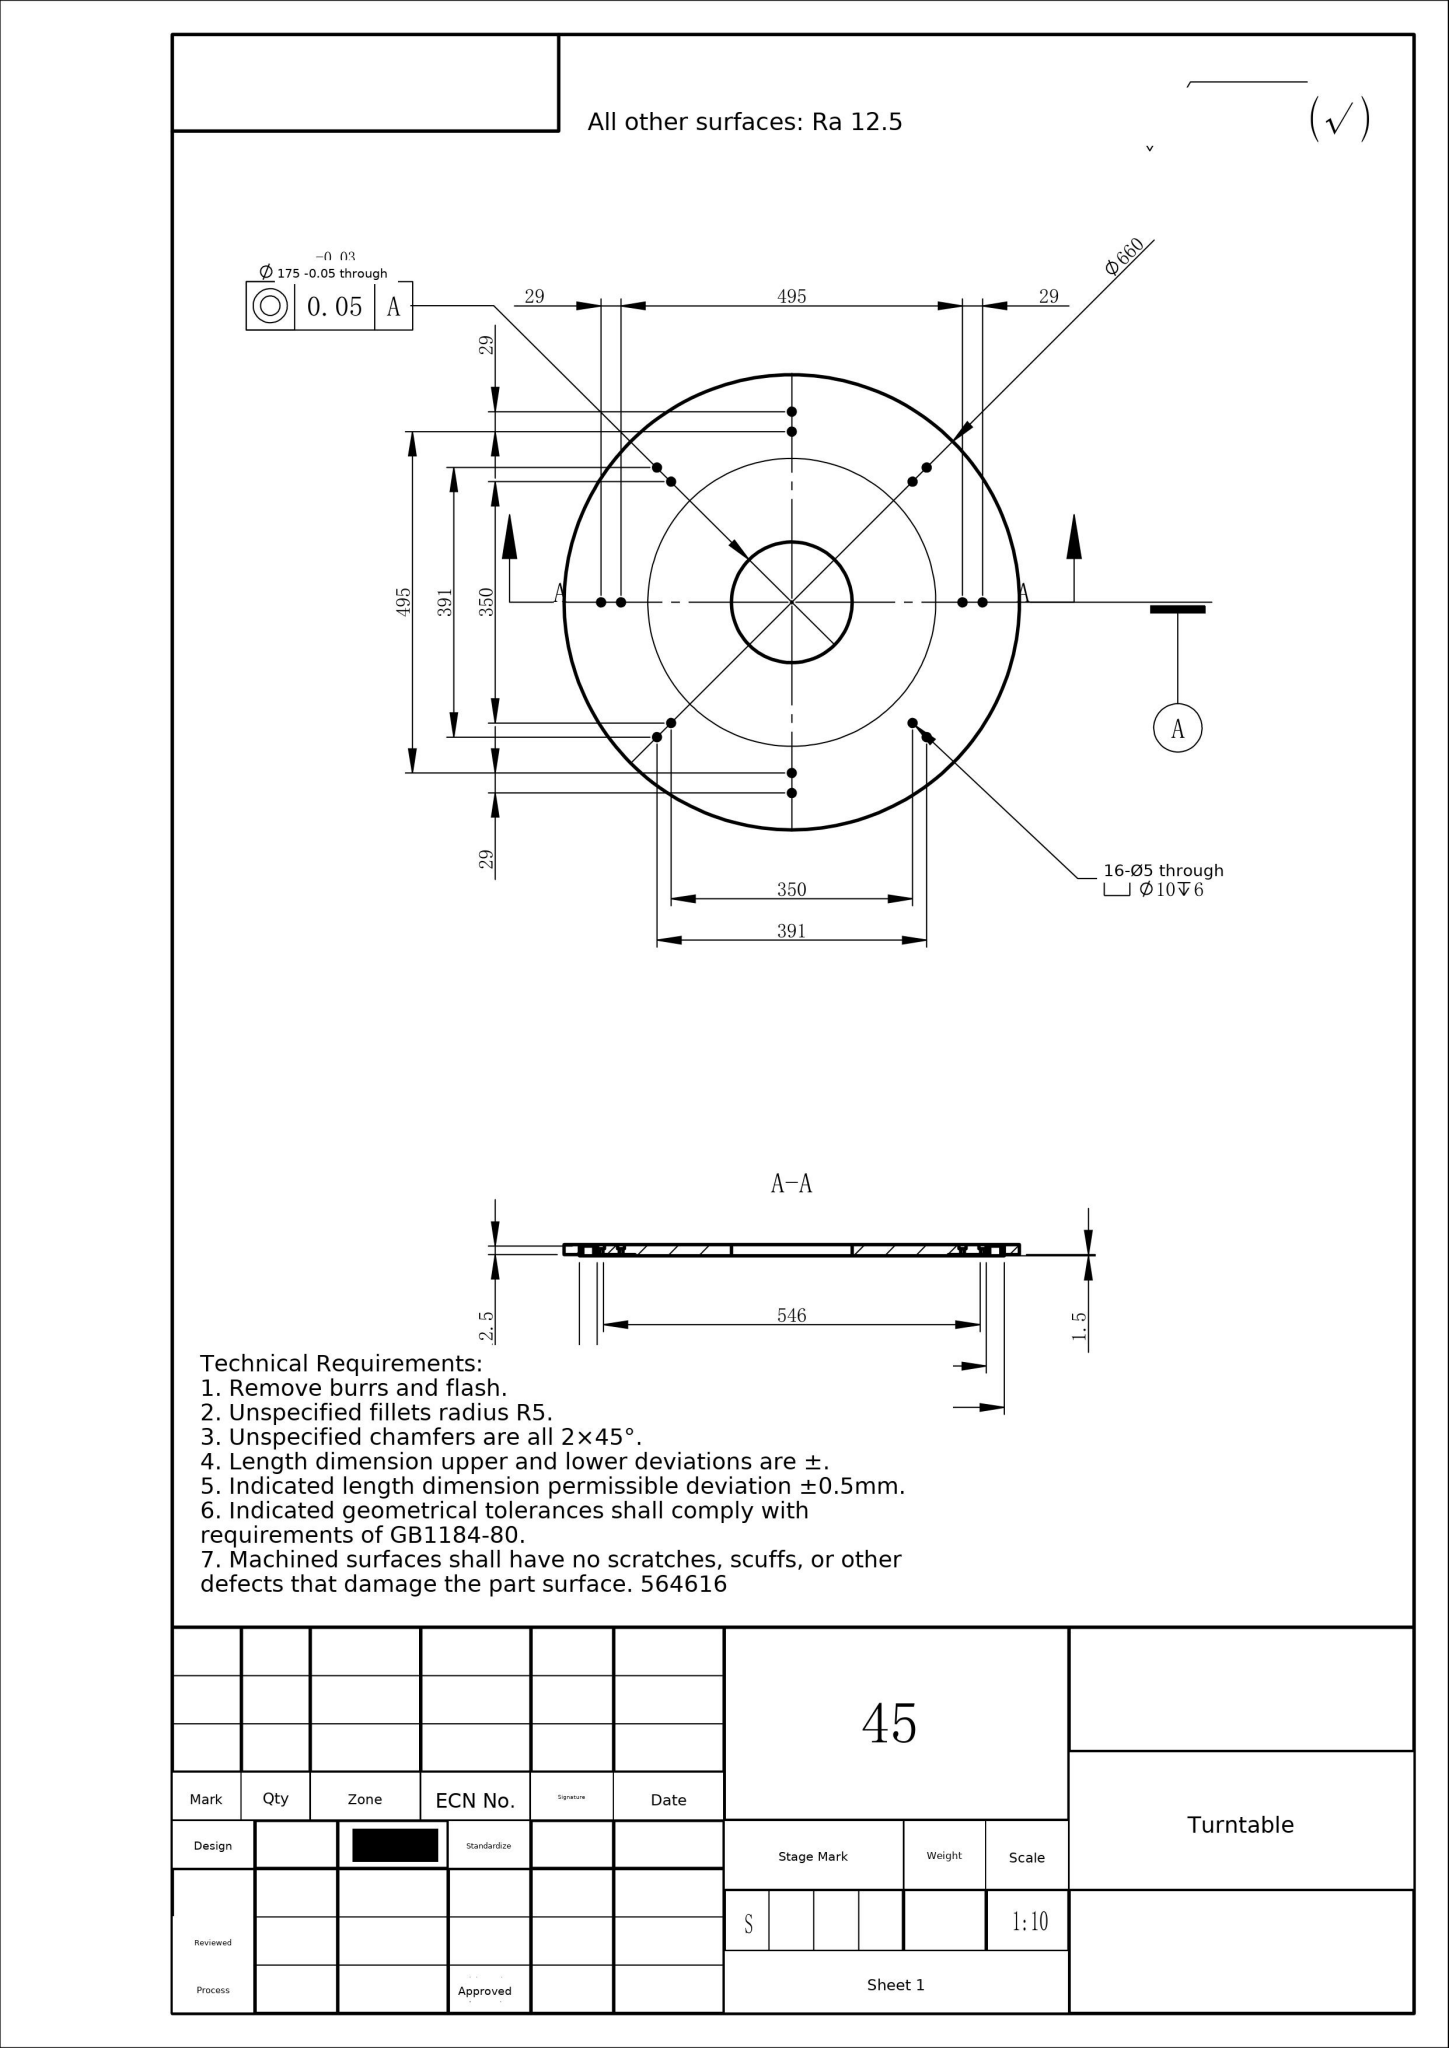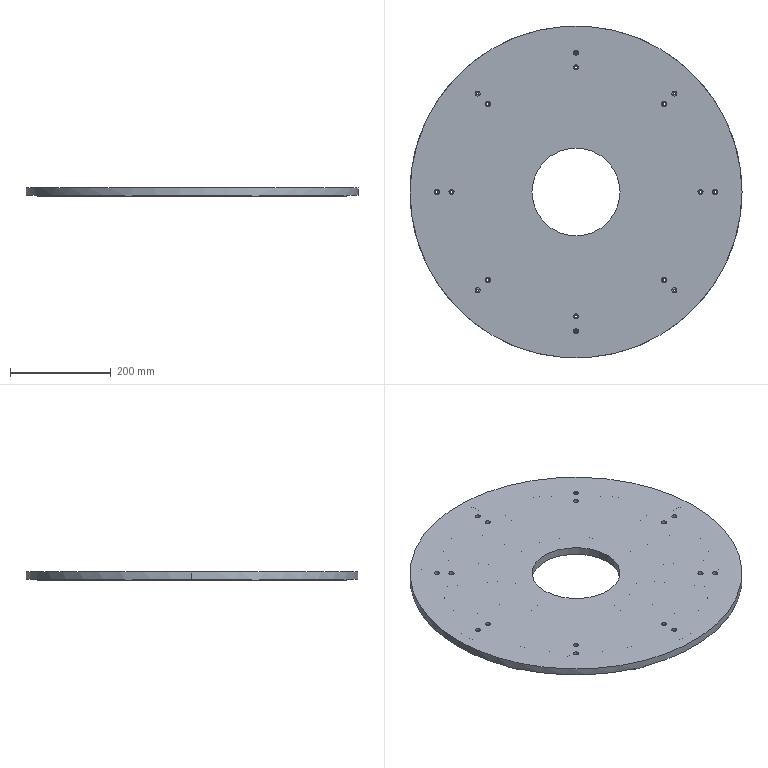Part | SolidWorks | drawing in inches | material 45 | 1 solid | 451 faces | box 660 x 660 x 16 mm | volume 3456434 mm3 | cylinder 241 | plane 162 | cone 48 | commonest cylinder face diameters 10 x68 2.5 x48 20 x40 5.3 x32 9 x22 12 x11 250 x8 550 x8